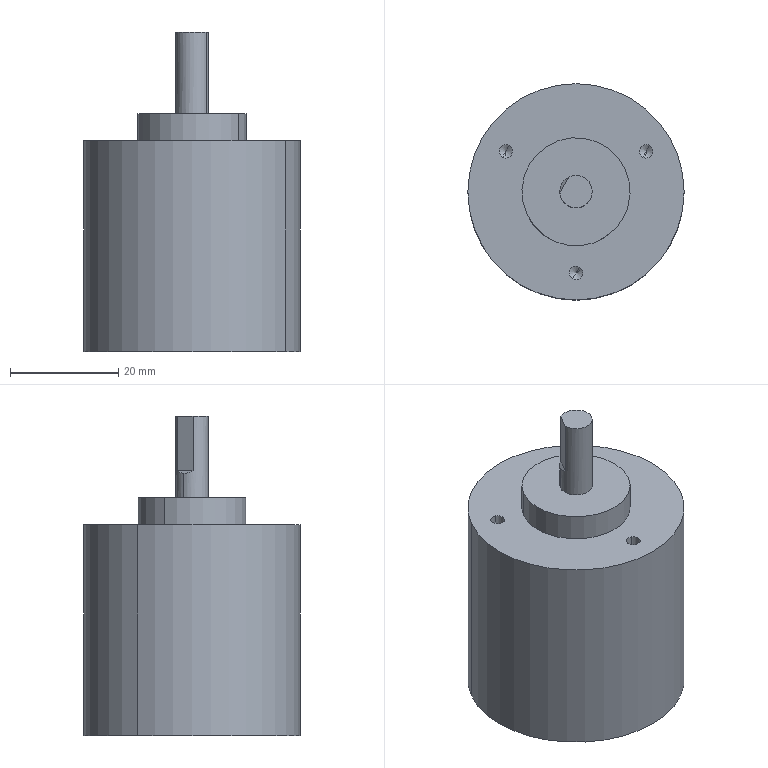Component | SolidWorks | 12AEncoder-1 | 1 solid | 24 faces | box 40 x 40 x 59 mm | volume 50878 mm3 | cylinder 12 | cone 6 | plane 6 | commonest cylinder face diameters 2.5 x6 40 x2 20 x2 6 x2
build123d program:
from build123d import *

# Parameters (mm, degrees)
CUT_EXTRUDE1_DEPTH    = 5
M3_TAPPED_HOLE1_D     = 2.5
M3_TAPPED_HOLE1_DEPTH = 7.5
M3_TAPPED_HOLE1_TIP   = 0.7511


with BuildPart() as part:
    # Sketch1 → Revolve1 (revolve)
    with BuildSketch(Plane.XY):
        Polygon((0, 0), (0, 3), (15, 3), (15, 10), (20, 10), (20, 20), (59, 20), (59, 0), align=None)
    revolve(axis=Axis((59, 0, 0), (-1, 0, 0)))

    # Sketch2 → Cut-Extrude1 (cut, symmetric)
    with BuildSketch(Plane.XY):
        Polygon((0, 2.5), (10, 2.5), (11.688, 4.188), (0, 4.188), align=None)
    extrude(amount=CUT_EXTRUDE1_DEPTH, both=True, mode=Mode.SUBTRACT)

    # M3 Tapped Hole1
    with Locations(Plane(origin=(20, 15, 0), x_dir=(0, -1, 0), z_dir=(-1, 0, 0))):
        with Locations((0, 0), (22.5, 12.99), (22.5, -12.99)):
            Hole(M3_TAPPED_HOLE1_D / 2, depth=M3_TAPPED_HOLE1_DEPTH)
            with Locations((0, 0, -(M3_TAPPED_HOLE1_DEPTH + M3_TAPPED_HOLE1_TIP / 2))):  # 118° drill point
                Cone(0, M3_TAPPED_HOLE1_D / 2, M3_TAPPED_HOLE1_TIP, mode=Mode.SUBTRACT)


solid = part.part

# Placed as in the assembly
solid = solid.moved(Location((120.894, 57.671, -106.26), (-90, 30, 90)))
STEP:
#1=COLOUR_RGB('',0.7922,0.8196,0.9333);
#2=FILL_AREA_STYLE_COLOUR('',#1);
#3=FILL_AREA_STYLE('',(#2));
#4=SURFACE_STYLE_FILL_AREA(#3);
#5=SURFACE_SIDE_STYLE('',(#4));
#6=SURFACE_STYLE_USAGE(.BOTH.,#5);
#7=PRESENTATION_STYLE_ASSIGNMENT((#6));
#8=CARTESIAN_POINT('',(4.224,2.523,-5.266));
#9=VERTEX_POINT('',#8);
#10=CARTESIAN_POINT('',(4.273,2.608,-5.266));
#11=VERTEX_POINT('',#10);
#12=CARTESIAN_POINT('',(4.248,2.566,-5.266));
#13=DIRECTION('',(-0.,0.,1.));
#14=DIRECTION('',(0.5,0.866,0.));
#15=AXIS2_PLACEMENT_3D('',#12,#13,#14);
#16=CIRCLE('',#15,0.04921);
#17=EDGE_CURVE('',#9,#11,#16,.T.);
#18=ORIENTED_EDGE('',*,*,#17,.F.);
#19=CARTESIAN_POINT('',(4.224,2.523,-4.971));
#20=VERTEX_POINT('',#19);
#21=CARTESIAN_POINT('',(4.224,2.523,-4.971));
#22=DIRECTION('',(-0.,0.,1.));
#23=VECTOR('',#22,39.37);
#24=LINE('',#21,#23);
#25=EDGE_CURVE('',#9,#20,#24,.T.);
#26=ORIENTED_EDGE('',*,*,#25,.T.);
#27=CARTESIAN_POINT('',(4.273,2.608,-4.971));
#28=VERTEX_POINT('',#27);
#29=CARTESIAN_POINT('',(4.248,2.566,-4.971));
#30=DIRECTION('',(-0.,0.,1.));
#31=DIRECTION('',(0.5,0.866,0.));
#32=AXIS2_PLACEMENT_3D('',#29,#30,#31);
#33=CIRCLE('',#32,0.04921);
#34=EDGE_CURVE('',#20,#28,#33,.T.);
#35=ORIENTED_EDGE('',*,*,#34,.T.);
#36=CARTESIAN_POINT('',(4.273,2.608,-4.971));
#37=DIRECTION('',(-0.,0.,1.));
#38=VECTOR('',#37,39.37);
#39=LINE('',#36,#38);
#40=EDGE_CURVE('',#11,#28,#39,.T.);
#41=ORIENTED_EDGE('',*,*,#40,.F.);
#42=EDGE_LOOP('',(#18,#26,#35,#41));
#43=FACE_OUTER_BOUND('',#42,.T.);
#44=CARTESIAN_POINT('',(4.248,2.566,-4.971));
#45=DIRECTION('',(-0.,0.,1.));
#46=DIRECTION('',(0.5,0.866,0.));
#47=AXIS2_PLACEMENT_3D('',#44,#45,#46);
#48=CYLINDRICAL_SURFACE('',#47,0.04921);
#49=ADVANCED_FACE('',(#43),#48,.F.);
#50=CARTESIAN_POINT('',(4.248,2.566,-5.296));
#51=VERTEX_POINT('',#50);
#52=CARTESIAN_POINT('',(4.273,2.608,-5.266));
#53=DIRECTION('',(0.4286,0.7423,0.515));
#54=VECTOR('',#53,39.37);
#55=LINE('',#52,#54);
#56=EDGE_CURVE('',#51,#11,#55,.T.);
#57=ORIENTED_EDGE('',*,*,#56,.F.);
#58=CARTESIAN_POINT('',(4.224,2.523,-5.266));
#59=DIRECTION('',(-0.4286,-0.7423,0.515));
#60=VECTOR('',#59,39.37);
#61=LINE('',#58,#60);
#62=EDGE_CURVE('',#51,#9,#61,.T.);
#63=ORIENTED_EDGE('',*,*,#62,.T.);
#64=ORIENTED_EDGE('',*,*,#17,.T.);
#65=EDGE_LOOP('',(#57,#63,#64));
#66=FACE_OUTER_BOUND('',#65,.T.);
#67=CARTESIAN_POINT('',(4.248,2.566,-5.266));
#68=DIRECTION('',(-0.,0.,1.));
#69=DIRECTION('',(0.5,0.866,0.));
#70=AXIS2_PLACEMENT_3D('',#67,#68,#69);
#71=CONICAL_SURFACE('',#70,0.04921,1.03);
#72=ADVANCED_FACE('',(#66),#71,.F.);
#73=CARTESIAN_POINT('',(5.246,2.523,-5.266));
#74=VERTEX_POINT('',#73);
#75=CARTESIAN_POINT('',(5.296,2.608,-5.266));
#76=VERTEX_POINT('',#75);
#77=CARTESIAN_POINT('',(5.271,2.566,-5.266));
#78=DIRECTION('',(-0.,0.,1.));
#79=DIRECTION('',(0.5,0.866,0.));
#80=AXIS2_PLACEMENT_3D('',#77,#78,#79);
#81=CIRCLE('',#80,0.04921);
#82=EDGE_CURVE('',#74,#76,#81,.T.);
#83=ORIENTED_EDGE('',*,*,#82,.F.);
#84=CARTESIAN_POINT('',(5.246,2.523,-4.971));
#85=VERTEX_POINT('',#84);
#86=CARTESIAN_POINT('',(5.246,2.523,-4.971));
#87=DIRECTION('',(-0.,0.,1.));
#88=VECTOR('',#87,39.37);
#89=LINE('',#86,#88);
#90=EDGE_CURVE('',#74,#85,#89,.T.);
#91=ORIENTED_EDGE('',*,*,#90,.T.);
#92=CARTESIAN_POINT('',(5.296,2.608,-4.971));
#93=VERTEX_POINT('',#92);
#94=CARTESIAN_POINT('',(5.271,2.566,-4.971));
#95=DIRECTION('',(-0.,0.,1.));
#96=DIRECTION('',(0.5,0.866,0.));
#97=AXIS2_PLACEMENT_3D('',#94,#95,#96);
#98=CIRCLE('',#97,0.04921);
#99=EDGE_CURVE('',#85,#93,#98,.T.);
#100=ORIENTED_EDGE('',*,*,#99,.T.);
#101=CARTESIAN_POINT('',(5.296,2.608,-4.971));
#102=DIRECTION('',(-0.,0.,1.));
#103=VECTOR('',#102,39.37);
#104=LINE('',#101,#103);
#105=EDGE_CURVE('',#76,#93,#104,.T.);
#106=ORIENTED_EDGE('',*,*,#105,.F.);
#107=EDGE_LOOP('',(#83,#91,#100,#106));
#108=FACE_OUTER_BOUND('',#107,.T.);
#109=CARTESIAN_POINT('',(5.271,2.566,-4.971));
#110=DIRECTION('',(-0.,0.,1.));
#111=DIRECTION('',(0.5,0.866,0.));
#112=AXIS2_PLACEMENT_3D('',#109,#110,#111);
#113=CYLINDRICAL_SURFACE('',#112,0.04921);
#114=ADVANCED_FACE('',(#108),#113,.F.);
#115=CARTESIAN_POINT('',(5.271,2.566,-5.296));
#116=VERTEX_POINT('',#115);
#117=CARTESIAN_POINT('',(5.296,2.608,-5.266));
#118=DIRECTION('',(0.4286,0.7423,0.515));
#119=VECTOR('',#118,39.37);
#120=LINE('',#117,#119);
#121=EDGE_CURVE('',#116,#76,#120,.T.);
#122=ORIENTED_EDGE('',*,*,#121,.F.);
#123=CARTESIAN_POINT('',(5.246,2.523,-5.266));
#124=DIRECTION('',(-0.4286,-0.7423,0.515));
#125=VECTOR('',#124,39.37);
#126=LINE('',#123,#125);
#127=EDGE_CURVE('',#116,#74,#126,.T.);
#128=ORIENTED_EDGE('',*,*,#127,.T.);
#129=ORIENTED_EDGE('',*,*,#82,.T.);
#130=EDGE_LOOP('',(#122,#128,#129));
#131=FACE_OUTER_BOUND('',#130,.T.);
#132=CARTESIAN_POINT('',(5.271,2.566,-5.266));
#133=DIRECTION('',(-0.,0.,1.));
#134=DIRECTION('',(0.5,0.866,0.));
#135=AXIS2_PLACEMENT_3D('',#132,#133,#134);
#136=CONICAL_SURFACE('',#135,0.04921,1.03);
#137=ADVANCED_FACE('',(#131),#136,.F.);
#138=CARTESIAN_POINT('',(4.735,1.637,-5.266));
#139=VERTEX_POINT('',#138);
#140=CARTESIAN_POINT('',(4.784,1.723,-5.266));
#141=VERTEX_POINT('',#140);
#142=CARTESIAN_POINT('',(4.76,1.68,-5.266));
#143=DIRECTION('',(-0.,0.,1.));
#144=DIRECTION('',(0.5,0.866,0.));
#145=AXIS2_PLACEMENT_3D('',#142,#143,#144);
#146=CIRCLE('',#145,0.04921);
#147=EDGE_CURVE('',#139,#141,#146,.T.);
#148=ORIENTED_EDGE('',*,*,#147,.F.);
#149=CARTESIAN_POINT('',(4.735,1.637,-4.971));
#150=VERTEX_POINT('',#149);
#151=CARTESIAN_POINT('',(4.735,1.637,-4.971));
#152=DIRECTION('',(-0.,0.,1.));
#153=VECTOR('',#152,39.37);
#154=LINE('',#151,#153);
#155=EDGE_CURVE('',#139,#150,#154,.T.);
#156=ORIENTED_EDGE('',*,*,#155,.T.);
#157=CARTESIAN_POINT('',(4.784,1.723,-4.971));
#158=VERTEX_POINT('',#157);
#159=CARTESIAN_POINT('',(4.76,1.68,-4.971));
#160=DIRECTION('',(-0.,0.,1.));
#161=DIRECTION('',(0.5,0.866,0.));
#162=AXIS2_PLACEMENT_3D('',#159,#160,#161);
#163=CIRCLE('',#162,0.04921);
#164=EDGE_CURVE('',#150,#158,#163,.T.);
#165=ORIENTED_EDGE('',*,*,#164,.T.);
#166=CARTESIAN_POINT('',(4.784,1.723,-4.971));
#167=DIRECTION('',(-0.,0.,1.));
#168=VECTOR('',#167,39.37);
#169=LINE('',#166,#168);
#170=EDGE_CURVE('',#141,#158,#169,.T.);
#171=ORIENTED_EDGE('',*,*,#170,.F.);
#172=EDGE_LOOP('',(#148,#156,#165,#171));
#173=FACE_OUTER_BOUND('',#172,.T.);
#174=CARTESIAN_POINT('',(4.76,1.68,-4.971));
#175=DIRECTION('',(-0.,0.,1.));
#176=DIRECTION('',(0.5,0.866,0.));
#177=AXIS2_PLACEMENT_3D('',#174,#175,#176);
#178=CYLINDRICAL_SURFACE('',#177,0.04921);
#179=ADVANCED_FACE('',(#173),#178,.F.);
#180=CARTESIAN_POINT('',(4.76,1.68,-5.296));
#181=VERTEX_POINT('',#180);
#182=CARTESIAN_POINT('',(4.784,1.723,-5.266));
#183=DIRECTION('',(0.4286,0.7423,0.515));
#184=VECTOR('',#183,39.37);
#185=LINE('',#182,#184);
#186=EDGE_CURVE('',#181,#141,#185,.T.);
#187=ORIENTED_EDGE('',*,*,#186,.F.);
#188=CARTESIAN_POINT('',(4.735,1.637,-5.266));
#189=DIRECTION('',(-0.4286,-0.7423,0.515));
#190=VECTOR('',#189,39.37);
#191=LINE('',#188,#190);
#192=EDGE_CURVE('',#181,#139,#191,.T.);
#193=ORIENTED_EDGE('',*,*,#192,.T.);
#194=ORIENTED_EDGE('',*,*,#147,.T.);
#195=EDGE_LOOP('',(#187,#193,#194));
#196=FACE_OUTER_BOUND('',#195,.T.);
#197=CARTESIAN_POINT('',(4.76,1.68,-5.266));
#198=DIRECTION('',(-0.,0.,1.));
#199=DIRECTION('',(0.5,0.866,0.));
#200=AXIS2_PLACEMENT_3D('',#197,#198,#199);
#201=CONICAL_SURFACE('',#200,0.04921,1.03);
#202=ADVANCED_FACE('',(#196),#201,.F.);
#203=CARTESIAN_POINT('',(4.078,2.664,-4.971));
#204=VERTEX_POINT('',#203);
#205=CARTESIAN_POINT('',(5.442,1.877,-4.971));
#206=VERTEX_POINT('',#205);
#207=CARTESIAN_POINT('',(4.76,2.271,-4.971));
#208=DIRECTION('',(-0.,-0.,-1.));
#209=DIRECTION('',(-0.866,0.5,0.));
#210=AXIS2_PLACEMENT_3D('',#207,#208,#209);
#211=CIRCLE('',#210,0.7874);
#212=EDGE_CURVE('',#204,#206,#211,.T.);
#213=ORIENTED_EDGE('',*,*,#212,.T.);
#214=CARTESIAN_POINT('',(5.442,1.877,-6.506));
#215=VERTEX_POINT('',#214);
#216=CARTESIAN_POINT('',(5.442,1.877,-6.506));
#217=DIRECTION('',(-0.,-0.,-1.));
#218=VECTOR('',#217,39.37);
#219=LINE('',#216,#218);
#220=EDGE_CURVE('',#206,#215,#219,.T.);
#221=ORIENTED_EDGE('',*,*,#220,.T.);
#222=CARTESIAN_POINT('',(4.078,2.664,-6.506));
#223=VERTEX_POINT('',#222);
#224=CARTESIAN_POINT('',(4.76,2.271,-6.506));
#225=DIRECTION('',(-0.,-0.,-1.));
#226=DIRECTION('',(-0.866,0.5,0.));
#227=AXIS2_PLACEMENT_3D('',#224,#225,#226);
#228=CIRCLE('',#227,0.7874);
#229=EDGE_CURVE('',#223,#215,#228,.T.);
#230=ORIENTED_EDGE('',*,*,#229,.F.);
#231=CARTESIAN_POINT('',(4.078,2.664,-6.506));
#232=DIRECTION('',(-0.,-0.,-1.));
#233=VECTOR('',#232,39.37);
#234=LINE('',#231,#233);
#235=EDGE_CURVE('',#204,#223,#234,.T.);
#236=ORIENTED_EDGE('',*,*,#235,.F.);
#237=EDGE_LOOP('',(#213,#221,#230,#236));
#238=FACE_OUTER_BOUND('',#237,.T.);
#239=CARTESIAN_POINT('',(4.76,2.271,-6.506));
#240=DIRECTION('',(-0.,-0.,-1.));
#241=DIRECTION('',(-0.866,0.5,0.));
#242=AXIS2_PLACEMENT_3D('',#239,#240,#241);
#243=CYLINDRICAL_SURFACE('',#242,0.7874);
#244=ADVANCED_FACE('',(#238),#243,.T.);
#245=CARTESIAN_POINT('',(4.419,2.467,-4.774));
#246=VERTEX_POINT('',#245);
#247=CARTESIAN_POINT('',(5.101,2.074,-4.774));
#248=VERTEX_POINT('',#247);
#249=CARTESIAN_POINT('',(4.76,2.271,-4.774));
#250=DIRECTION('',(-0.,-0.,-1.));
#251=DIRECTION('',(-0.866,0.5,0.));
#252=AXIS2_PLACEMENT_3D('',#249,#250,#251);
#253=CIRCLE('',#252,0.3937);
#254=EDGE_CURVE('',#246,#248,#253,.T.);
#255=ORIENTED_EDGE('',*,*,#254,.T.);
#256=CARTESIAN_POINT('',(5.101,2.074,-4.971));
#257=VERTEX_POINT('',#256);
#258=CARTESIAN_POINT('',(5.101,2.074,-6.506));
#259=DIRECTION('',(-0.,-0.,-1.));
#260=VECTOR('',#259,39.37);
#261=LINE('',#258,#260);
#262=EDGE_CURVE('',#248,#257,#261,.T.);
#263=ORIENTED_EDGE('',*,*,#262,.T.);
#264=CARTESIAN_POINT('',(4.419,2.467,-4.971));
#265=VERTEX_POINT('',#264);
#266=CARTESIAN_POINT('',(4.76,2.271,-4.971));
#267=DIRECTION('',(-0.,-0.,-1.));
#268=DIRECTION('',(-0.866,0.5,0.));
#269=AXIS2_PLACEMENT_3D('',#266,#267,#268);
#270=CIRCLE('',#269,0.3937);
#271=EDGE_CURVE('',#265,#257,#270,.T.);
#272=ORIENTED_EDGE('',*,*,#271,.F.);
#273=CARTESIAN_POINT('',(4.419,2.467,-6.506));
#274=DIRECTION('',(-0.,-0.,-1.));
#275=VECTOR('',#274,39.37);
#276=LINE('',#273,#275);
#277=EDGE_CURVE('',#246,#265,#276,.T.);
#278=ORIENTED_EDGE('',*,*,#277,.F.);
#279=EDGE_LOOP('',(#255,#263,#272,#278));
#280=FACE_OUTER_BOUND('',#279,.T.);
#281=CARTESIAN_POINT('',(4.76,2.271,-6.506));
#282=DIRECTION('',(-0.,-0.,-1.));
#283=DIRECTION('',(-0.866,0.5,0.));
#284=AXIS2_PLACEMENT_3D('',#281,#282,#283);
#285=CYLINDRICAL_SURFACE('',#284,0.3937);
#286=ADVANCED_FACE('',(#280),#285,.T.);
#287=CARTESIAN_POINT('',(4.707,2.376,-4.183));
#288=VERTEX_POINT('',#287);
#289=CARTESIAN_POINT('',(4.862,2.211,-4.183));
#290=VERTEX_POINT('',#289);
#291=CARTESIAN_POINT('',(4.76,2.271,-4.183));
#292=DIRECTION('',(-0.,-0.,-1.));
#293=DIRECTION('',(-0.866,0.5,0.));
#294=AXIS2_PLACEMENT_3D('',#291,#292,#293);
#295=CIRCLE('',#294,0.1181);
#296=EDGE_CURVE('',#288,#290,#295,.T.);
#297=ORIENTED_EDGE('',*,*,#296,.T.);
#298=CARTESIAN_POINT('',(4.862,2.211,-4.774));
#299=VERTEX_POINT('',#298);
#300=CARTESIAN_POINT('',(4.862,2.211,-6.506));
#301=DIRECTION('',(-0.,-0.,-1.));
#302=VECTOR('',#301,39.37);
#303=LINE('',#300,#302);
#304=EDGE_CURVE('',#290,#299,#303,.T.);
#305=ORIENTED_EDGE('',*,*,#304,.T.);
#306=CARTESIAN_POINT('',(4.657,2.33,-4.774));
#307=VERTEX_POINT('',#306);
#308=CARTESIAN_POINT('',(4.76,2.271,-4.774));
#309=DIRECTION('',(-0.,-0.,-1.));
#310=DIRECTION('',(-0.866,0.5,0.));
#311=AXIS2_PLACEMENT_3D('',#308,#309,#310);
#312=CIRCLE('',#311,0.1181);
#313=EDGE_CURVE('',#307,#299,#312,.T.);
#314=ORIENTED_EDGE('',*,*,#313,.F.);
#315=CARTESIAN_POINT('',(4.657,2.33,-4.597));
#316=VERTEX_POINT('',#315);
#317=CARTESIAN_POINT('',(4.657,2.33,-6.506));
#318=DIRECTION('',(-0.,-0.,-1.));
#319=VECTOR('',#318,39.37);
#320=LINE('',#317,#319);
#321=EDGE_CURVE('',#316,#307,#320,.T.);
#322=ORIENTED_EDGE('',*,*,#321,.F.);
#323=CARTESIAN_POINT('',(4.707,2.376,-4.577));
#324=VERTEX_POINT('',#323);
#325=CARTESIAN_POINT('',(4.707,2.376,-4.577));
#326=CARTESIAN_POINT('',(4.686,2.366,-4.59));
#327=CARTESIAN_POINT('',(4.669,2.35,-4.597));
#328=CARTESIAN_POINT('',(4.657,2.33,-4.597));
#329=(BOUNDED_CURVE()B_SPLINE_CURVE(3,(#325,#326,#327,#328),.UNSPECIFIED.,.F.,.F.)B_SPLINE_CURVE_WITH_KNOTS((4,4),(5.697,6.283),.UNSPECIFIED.)CURVE()GEOMETRIC_REPRESENTATION_ITEM()RATIONAL_B_SPLINE_CURVE((1.,0.9716,0.9716,1.))REPRESENTATION_ITEM(''));
#330=EDGE_CURVE('',#324,#316,#329,.T.);
#331=ORIENTED_EDGE('',*,*,#330,.F.);
#332=CARTESIAN_POINT('',(4.707,2.376,-6.506));
#333=DIRECTION('',(-0.,-0.,-1.));
#334=VECTOR('',#333,39.37);
#335=LINE('',#332,#334);
#336=EDGE_CURVE('',#288,#324,#335,.T.);
#337=ORIENTED_EDGE('',*,*,#336,.F.);
#338=EDGE_LOOP('',(#297,#305,#314,#322,#331,#337));
#339=FACE_OUTER_BOUND('',#338,.T.);
#340=CARTESIAN_POINT('',(4.76,2.271,-6.506));
#341=DIRECTION('',(-0.,-0.,-1.));
#342=DIRECTION('',(-0.866,0.5,0.));
#343=AXIS2_PLACEMENT_3D('',#340,#341,#342);
#344=CYLINDRICAL_SURFACE('',#343,0.1181);
#345=ADVANCED_FACE('',(#339),#344,.T.);
#346=CARTESIAN_POINT('',(4.642,2.263,-4.183));
#347=VERTEX_POINT('',#346);
#348=CARTESIAN_POINT('',(4.576,2.149,-4.183));
#349=DIRECTION('',(0.5,0.866,-0.));
#350=VECTOR('',#349,39.37);
#351=LINE('',#348,#350);
#352=EDGE_CURVE('',#347,#288,#351,.T.);
#353=ORIENTED_EDGE('',*,*,#352,.F.);
#354=CARTESIAN_POINT('',(4.76,2.271,-4.183));
#355=DIRECTION('',(-0.,-0.,-1.));
#356=DIRECTION('',(-0.866,0.5,0.));
#357=AXIS2_PLACEMENT_3D('',#354,#355,#356);
#358=CIRCLE('',#357,0.1181);
#359=EDGE_CURVE('',#290,#347,#358,.T.);
#360=ORIENTED_EDGE('',*,*,#359,.F.);
#361=ORIENTED_EDGE('',*,*,#296,.F.);
#362=EDGE_LOOP('',(#353,#360,#361));
#363=FACE_OUTER_BOUND('',#362,.T.);
#364=CARTESIAN_POINT('',(4.76,2.271,-4.183));
#365=DIRECTION('',(0.,0.,1.));
#366=DIRECTION('',(0.866,-0.5,-0.));
#367=AXIS2_PLACEMENT_3D('',#364,#365,#366);
#368=PLANE('',#367);
#369=ADVANCED_FACE('',(#363),#368,.T.);
#370=ORIENTED_EDGE('',*,*,#304,.F.);
#371=ORIENTED_EDGE('',*,*,#359,.T.);
#372=CARTESIAN_POINT('',(4.642,2.263,-4.577));
#373=VERTEX_POINT('',#372);
#374=CARTESIAN_POINT('',(4.642,2.263,-6.506));
#375=DIRECTION('',(0.,0.,1.));
#376=VECTOR('',#375,39.37);
#377=LINE('',#374,#376);
#378=EDGE_CURVE('',#373,#347,#377,.T.);
#379=ORIENTED_EDGE('',*,*,#378,.F.);
#380=CARTESIAN_POINT('',(4.657,2.33,-4.597));
#381=CARTESIAN_POINT('',(4.646,2.309,-4.597));
#382=CARTESIAN_POINT('',(4.64,2.287,-4.59));
#383=CARTESIAN_POINT('',(4.642,2.263,-4.577));
#384=(BOUNDED_CURVE()B_SPLINE_CURVE(3,(#380,#381,#382,#383),.UNSPECIFIED.,.F.,.F.)B_SPLINE_CURVE_WITH_KNOTS((4,4),(0.,0.5857),.UNSPECIFIED.)CURVE()GEOMETRIC_REPRESENTATION_ITEM()RATIONAL_B_SPLINE_CURVE((1.,0.9716,0.9716,1.))REPRESENTATION_ITEM(''));
#385=EDGE_CURVE('',#316,#373,#384,.T.);
#386=ORIENTED_EDGE('',*,*,#385,.F.);
#387=ORIENTED_EDGE('',*,*,#321,.T.);
#388=CARTESIAN_POINT('',(4.76,2.271,-4.774));
#389=DIRECTION('',(-0.,-0.,-1.));
#390=DIRECTION('',(-0.866,0.5,0.));
#391=AXIS2_PLACEMENT_3D('',#388,#389,#390);
#392=CIRCLE('',#391,0.1181);
#393=EDGE_CURVE('',#299,#307,#392,.T.);
#394=ORIENTED_EDGE('',*,*,#393,.F.);
#395=EDGE_LOOP('',(#370,#371,#379,#386,#387,#394));
#396=FACE_OUTER_BOUND('',#395,.T.);
#397=CARTESIAN_POINT('',(4.76,2.271,-6.506));
#398=DIRECTION('',(-0.,-0.,-1.));
#399=DIRECTION('',(-0.866,0.5,0.));
#400=AXIS2_PLACEMENT_3D('',#397,#398,#399);
#401=CYLINDRICAL_SURFACE('',#400,0.1181);
#402=ADVANCED_FACE('',(#396),#401,.T.);
#403=ORIENTED_EDGE('',*,*,#313,.T.);
#404=ORIENTED_EDGE('',*,*,#393,.T.);
#405=EDGE_LOOP('',(#403,#404));
#406=FACE_BOUND('',#405,.T.);
#407=ORIENTED_EDGE('',*,*,#254,.F.);
#408=CARTESIAN_POINT('',(4.76,2.271,-4.774));
#409=DIRECTION('',(-0.,-0.,-1.));
#410=DIRECTION('',(-0.866,0.5,0.));
#411=AXIS2_PLACEMENT_3D('',#408,#409,#410);
#412=CIRCLE('',#411,0.3937);
#413=EDGE_CURVE('',#248,#246,#412,.T.);
#414=ORIENTED_EDGE('',*,*,#413,.F.);
#415=EDGE_LOOP('',(#407,#414));
#416=FACE_OUTER_BOUND('',#415,.T.);
#417=CARTESIAN_POINT('',(4.657,2.33,-4.774));
#418=DIRECTION('',(0.,0.,1.));
#419=DIRECTION('',(0.866,-0.5,-0.));
#420=AXIS2_PLACEMENT_3D('',#417,#418,#419);
#421=PLANE('',#420);
#422=ADVANCED_FACE('',(#406,#416),#421,.T.);
#423=ORIENTED_EDGE('',*,*,#262,.F.);
#424=ORIENTED_EDGE('',*,*,#413,.T.);
#425=ORIENTED_EDGE('',*,*,#277,.T.);
#426=CARTESIAN_POINT('',(4.76,2.271,-4.971));
#427=DIRECTION('',(-0.,-0.,-1.));
#428=DIRECTION('',(-0.866,0.5,0.));
#429=AXIS2_PLACEMENT_3D('',#426,#427,#428);
#430=CIRCLE('',#429,0.3937);
#431=EDGE_CURVE('',#257,#265,#430,.T.);
#432=ORIENTED_EDGE('',*,*,#431,.F.);
#433=EDGE_LOOP('',(#423,#424,#425,#432));
#434=FACE_OUTER_BOUND('',#433,.T.);
#435=CARTESIAN_POINT('',(4.76,2.271,-6.506));
#436=DIRECTION('',(-0.,-0.,-1.));
#437=DIRECTION('',(-0.866,0.5,0.));
#438=AXIS2_PLACEMENT_3D('',#435,#436,#437);
#439=CYLINDRICAL_SURFACE('',#438,0.3937);
#440=ADVANCED_FACE('',(#434),#439,.T.);
#441=CARTESIAN_POINT('',(4.248,2.566,-4.971));
#442=DIRECTION('',(-0.,0.,1.));
#443=DIRECTION('',(0.5,0.866,0.));
#444=AXIS2_PLACEMENT_3D('',#441,#442,#443);
#445=CIRCLE('',#444,0.04921);
#446=EDGE_CURVE('',#28,#20,#445,.T.);
#447=ORIENTED_EDGE('',*,*,#446,.F.);
#448=ORIENTED_EDGE('',*,*,#34,.F.);
#449=EDGE_LOOP('',(#447,#448));
#450=FACE_BOUND('',#449,.T.);
#451=CARTESIAN_POINT('',(5.271,2.566,-4.971));
#452=DIRECTION('',(-0.,0.,1.));
#453=DIRECTION('',(0.5,0.866,0.));
#454=AXIS2_PLACEMENT_3D('',#451,#452,#453);
#455=CIRCLE('',#454,0.04921);
#456=EDGE_CURVE('',#93,#85,#455,.T.);
#457=ORIENTED_EDGE('',*,*,#456,.F.);
#458=ORIENTED_EDGE('',*,*,#99,.F.);
#459=EDGE_LOOP('',(#457,#458));
#460=FACE_BOUND('',#459,.T.);
#461=CARTESIAN_POINT('',(4.76,1.68,-4.971));
#462=DIRECTION('',(-0.,0.,1.));
#463=DIRECTION('',(0.5,0.866,0.));
#464=AXIS2_PLACEMENT_3D('',#461,#462,#463);
#465=CIRCLE('',#464,0.04921);
#466=EDGE_CURVE('',#158,#150,#465,.T.);
#467=ORIENTED_EDGE('',*,*,#466,.F.);
#468=ORIENTED_EDGE('',*,*,#164,.F.);
#469=EDGE_LOOP('',(#467,#468));
#470=FACE_BOUND('',#469,.T.);
#471=ORIENTED_EDGE('',*,*,#271,.T.);
#472=ORIENTED_EDGE('',*,*,#431,.T.);
#473=EDGE_LOOP('',(#471,#472));
#474=FACE_BOUND('',#473,.T.);
#475=ORIENTED_EDGE('',*,*,#212,.F.);
#476=CARTESIAN_POINT('',(4.76,2.271,-4.971));
#477=DIRECTION('',(-0.,-0.,-1.));
#478=DIRECTION('',(-0.866,0.5,0.));
#479=AXIS2_PLACEMENT_3D('',#476,#477,#478);
#480=CIRCLE('',#479,0.7874);
#481=EDGE_CURVE('',#206,#204,#480,.T.);
#482=ORIENTED_EDGE('',*,*,#481,.F.);
#483=EDGE_LOOP('',(#475,#482));
#484=FACE_OUTER_BOUND('',#483,.T.);
#485=CARTESIAN_POINT('',(4.419,2.467,-4.971));
#486=DIRECTION('',(0.,0.,1.));
#487=DIRECTION('',(0.866,-0.5,-0.));
#488=AXIS2_PLACEMENT_3D('',#485,#486,#487);
#489=PLANE('',#488);
#490=ADVANCED_FACE('',(#450,#460,#470,#474,#484),#489,.T.);
#491=ORIENTED_EDGE('',*,*,#220,.F.);
#492=ORIENTED_EDGE('',*,*,#481,.T.);
#493=ORIENTED_EDGE('',*,*,#235,.T.);
#494=CARTESIAN_POINT('',(4.76,2.271,-6.506));
#495=DIRECTION('',(-0.,-0.,-1.));
#496=DIRECTION('',(-0.866,0.5,0.));
#497=AXIS2_PLACEMENT_3D('',#494,#495,#496);
#498=CIRCLE('',#497,0.7874);
#499=EDGE_CURVE('',#215,#223,#498,.T.);
#500=ORIENTED_EDGE('',*,*,#499,.F.);
#501=EDGE_LOOP('',(#491,#492,#493,#500));
#502=FACE_OUTER_BOUND('',#501,.T.);
#503=CARTESIAN_POINT('',(4.76,2.271,-6.506));
#504=DIRECTION('',(-0.,-0.,-1.));
#505=DIRECTION('',(-0.866,0.5,0.));
#506=AXIS2_PLACEMENT_3D('',#503,#504,#505);
#507=CYLINDRICAL_SURFACE('',#506,0.7874);
#508=ADVANCED_FACE('',(#502),#507,.T.);
#509=ORIENTED_EDGE('',*,*,#229,.T.);
#510=ORIENTED_EDGE('',*,*,#499,.T.);
#511=EDGE_LOOP('',(#509,#510));
#512=FACE_OUTER_BOUND('',#511,.T.);
#513=CARTESIAN_POINT('',(4.078,2.664,-6.506));
#514=DIRECTION('',(-0.,-0.,-1.));
#515=DIRECTION('',(-0.866,0.5,0.));
#516=AXIS2_PLACEMENT_3D('',#513,#514,#515);
#517=PLANE('',#516);
#518=ADVANCED_FACE('',(#512),#517,.T.);
#519=ORIENTED_EDGE('',*,*,#330,.T.);
#520=ORIENTED_EDGE('',*,*,#385,.T.);
#521=CARTESIAN_POINT('',(4.576,2.149,-4.577));
#522=DIRECTION('',(0.5,0.866,-0.));
#523=VECTOR('',#522,39.37);
#524=LINE('',#521,#523);
#525=EDGE_CURVE('',#373,#324,#524,.T.);
#526=ORIENTED_EDGE('',*,*,#525,.T.);
#527=EDGE_LOOP('',(#519,#520,#526));
#528=FACE_OUTER_BOUND('',#527,.T.);
#529=CARTESIAN_POINT('',(4.576,2.149,-4.577));
#530=DIRECTION('',(0.6124,-0.3536,-0.7071));
#531=DIRECTION('',(-0.6124,0.3536,-0.7071));
#532=AXIS2_PLACEMENT_3D('',#529,#530,#531);
#533=PLANE('',#532);
#534=ADVANCED_FACE('',(#528),#533,.F.);
#535=ORIENTED_EDGE('',*,*,#378,.T.);
#536=ORIENTED_EDGE('',*,*,#352,.T.);
#537=ORIENTED_EDGE('',*,*,#336,.T.);
#538=ORIENTED_EDGE('',*,*,#525,.F.);
#539=EDGE_LOOP('',(#535,#536,#537,#538));
#540=FACE_OUTER_BOUND('',#539,.T.);
#541=CARTESIAN_POINT('',(4.576,2.149,-4.183));
#542=DIRECTION('',(0.866,-0.5,0.));
#543=DIRECTION('',(-0.5,-0.866,0.));
#544=AXIS2_PLACEMENT_3D('',#541,#542,#543);
#545=PLANE('',#544);
#546=ADVANCED_FACE('',(#540),#545,.F.);
#547=ORIENTED_EDGE('',*,*,#192,.F.);
#548=ORIENTED_EDGE('',*,*,#186,.T.);
#549=CARTESIAN_POINT('',(4.76,1.68,-5.266));
#550=DIRECTION('',(-0.,0.,1.));
#551=DIRECTION('',(0.5,0.866,0.));
#552=AXIS2_PLACEMENT_3D('',#549,#550,#551);
#553=CIRCLE('',#552,0.04921);
#554=EDGE_CURVE('',#141,#139,#553,.T.);
#555=ORIENTED_EDGE('',*,*,#554,.T.);
#556=EDGE_LOOP('',(#547,#548,#555));
#557=FACE_OUTER_BOUND('',#556,.T.);
#558=CARTESIAN_POINT('',(4.76,1.68,-5.266));
#559=DIRECTION('',(-0.,0.,1.));
#560=DIRECTION('',(0.5,0.866,0.));
#561=AXIS2_PLACEMENT_3D('',#558,#559,#560);
#562=CONICAL_SURFACE('',#561,0.04921,1.03);
#563=ADVANCED_FACE('',(#557),#562,.F.);
#564=ORIENTED_EDGE('',*,*,#155,.F.);
#565=ORIENTED_EDGE('',*,*,#554,.F.);
#566=ORIENTED_EDGE('',*,*,#170,.T.);
#567=ORIENTED_EDGE('',*,*,#466,.T.);
#568=EDGE_LOOP('',(#564,#565,#566,#567));
#569=FACE_OUTER_BOUND('',#568,.T.);
#570=CARTESIAN_POINT('',(4.76,1.68,-4.971));
#571=DIRECTION('',(-0.,0.,1.));
#572=DIRECTION('',(0.5,0.866,0.));
#573=AXIS2_PLACEMENT_3D('',#570,#571,#572);
#574=CYLINDRICAL_SURFACE('',#573,0.04921);
#575=ADVANCED_FACE('',(#569),#574,.F.);
#576=ORIENTED_EDGE('',*,*,#127,.F.);
#577=ORIENTED_EDGE('',*,*,#121,.T.);
#578=CARTESIAN_POINT('',(5.271,2.566,-5.266));
#579=DIRECTION('',(-0.,0.,1.));
#580=DIRECTION('',(0.5,0.866,0.));
#581=AXIS2_PLACEMENT_3D('',#578,#579,#580);
#582=CIRCLE('',#581,0.04921);
#583=EDGE_CURVE('',#76,#74,#582,.T.);
#584=ORIENTED_EDGE('',*,*,#583,.T.);
#585=EDGE_LOOP('',(#576,#577,#584));
#586=FACE_OUTER_BOUND('',#585,.T.);
#587=CARTESIAN_POINT('',(5.271,2.566,-5.266));
#588=DIRECTION('',(-0.,0.,1.));
#589=DIRECTION('',(0.5,0.866,0.));
#590=AXIS2_PLACEMENT_3D('',#587,#588,#589);
#591=CONICAL_SURFACE('',#590,0.04921,1.03);
#592=ADVANCED_FACE('',(#586),#591,.F.);
#593=ORIENTED_EDGE('',*,*,#90,.F.);
#594=ORIENTED_EDGE('',*,*,#583,.F.);
#595=ORIENTED_EDGE('',*,*,#105,.T.);
#596=ORIENTED_EDGE('',*,*,#456,.T.);
#597=EDGE_LOOP('',(#593,#594,#595,#596));
#598=FACE_OUTER_BOUND('',#597,.T.);
#599=CARTESIAN_POINT('',(5.271,2.566,-4.971));
#600=DIRECTION('',(-0.,0.,1.));
#601=DIRECTION('',(0.5,0.866,0.));
#602=AXIS2_PLACEMENT_3D('',#599,#600,#601);
#603=CYLINDRICAL_SURFACE('',#602,0.04921);
#604=ADVANCED_FACE('',(#598),#603,.F.);
#605=ORIENTED_EDGE('',*,*,#62,.F.);
#606=ORIENTED_EDGE('',*,*,#56,.T.);
#607=CARTESIAN_POINT('',(4.248,2.566,-5.266));
#608=DIRECTION('',(-0.,0.,1.));
#609=DIRECTION('',(0.5,0.866,0.));
#610=AXIS2_PLACEMENT_3D('',#607,#608,#609);
#611=CIRCLE('',#610,0.04921);
#612=EDGE_CURVE('',#11,#9,#611,.T.);
#613=ORIENTED_EDGE('',*,*,#612,.T.);
#614=EDGE_LOOP('',(#605,#606,#613));
#615=FACE_OUTER_BOUND('',#614,.T.);
#616=CARTESIAN_POINT('',(4.248,2.566,-5.266));
#617=DIRECTION('',(-0.,0.,1.));
#618=DIRECTION('',(0.5,0.866,0.));
#619=AXIS2_PLACEMENT_3D('',#616,#617,#618);
#620=CONICAL_SURFACE('',#619,0.04921,1.03);
#621=ADVANCED_FACE('',(#615),#620,.F.);
#622=ORIENTED_EDGE('',*,*,#25,.F.);
#623=ORIENTED_EDGE('',*,*,#612,.F.);
#624=ORIENTED_EDGE('',*,*,#40,.T.);
#625=ORIENTED_EDGE('',*,*,#446,.T.);
#626=EDGE_LOOP('',(#622,#623,#624,#625));
#627=FACE_OUTER_BOUND('',#626,.T.);
#628=CARTESIAN_POINT('',(4.248,2.566,-4.971));
#629=DIRECTION('',(-0.,0.,1.));
#630=DIRECTION('',(0.5,0.866,0.));
#631=AXIS2_PLACEMENT_3D('',#628,#629,#630);
#632=CYLINDRICAL_SURFACE('',#631,0.04921);
#633=ADVANCED_FACE('',(#627),#632,.F.);
#634=CLOSED_SHELL('',(#49,#72,#114,#137,#179,#202,#244,#286,#345,#369,#402,#422,#440,#490,#508,#518,#534,#546,#563,#575,#592,#604,#621,#633));
#635=MANIFOLD_SOLID_BREP('',#634);
#636=STYLED_ITEM('',(#7),#635);
#637=(LENGTH_UNIT()NAMED_UNIT(*)SI_UNIT($,.METRE.));
#638=LENGTH_MEASURE_WITH_UNIT(LENGTH_MEASURE(0.0254),#637);
#639=DIMENSIONAL_EXPONENTS(1.,0.,0.,0.,0.,0.,0.);
#640=(CONVERSION_BASED_UNIT('',#638)LENGTH_UNIT()NAMED_UNIT(#639));
#641=UNCERTAINTY_MEASURE_WITH_UNIT(LENGTH_MEASURE(0.00001),#640,'','');
#642=(NAMED_UNIT(*)PLANE_ANGLE_UNIT()SI_UNIT($,.RADIAN.));
#643=(NAMED_UNIT(*)SI_UNIT($,.STERADIAN.)SOLID_ANGLE_UNIT());
#644=(GEOMETRIC_REPRESENTATION_CONTEXT(3)GLOBAL_UNCERTAINTY_ASSIGNED_CONTEXT((#641))GLOBAL_UNIT_ASSIGNED_CONTEXT((#640,#642,#643))REPRESENTATION_CONTEXT('',''));
#645=MECHANICAL_DESIGN_GEOMETRIC_PRESENTATION_REPRESENTATION('',(#636),#644);
#646=PRESENTATION_LAYER_ASSIGNMENT('','',(#636));
#647=CARTESIAN_POINT('',(0.,0.,0.));
#648=DIRECTION('',(0.,0.,1.));
#649=DIRECTION('',(1.,0.,0.));
#650=AXIS2_PLACEMENT_3D('',#647,#648,#649);
#651=(LENGTH_UNIT()NAMED_UNIT(*)SI_UNIT($,.METRE.));
#652=LENGTH_MEASURE_WITH_UNIT(LENGTH_MEASURE(0.0254),#651);
#653=DIMENSIONAL_EXPONENTS(1.,0.,0.,0.,0.,0.,0.);
#654=(CONVERSION_BASED_UNIT('',#652)LENGTH_UNIT()NAMED_UNIT(#653));
#655=UNCERTAINTY_MEASURE_WITH_UNIT(LENGTH_MEASURE(0.00001),#654,'','');
#656=(NAMED_UNIT(*)PLANE_ANGLE_UNIT()SI_UNIT($,.RADIAN.));
#657=(NAMED_UNIT(*)SI_UNIT($,.STERADIAN.)SOLID_ANGLE_UNIT());
#658=(GEOMETRIC_REPRESENTATION_CONTEXT(3)GLOBAL_UNCERTAINTY_ASSIGNED_CONTEXT((#655))GLOBAL_UNIT_ASSIGNED_CONTEXT((#654,#656,#657))REPRESENTATION_CONTEXT('',''));
#659=ADVANCED_BREP_SHAPE_REPRESENTATION('',(#635,#650),#658);